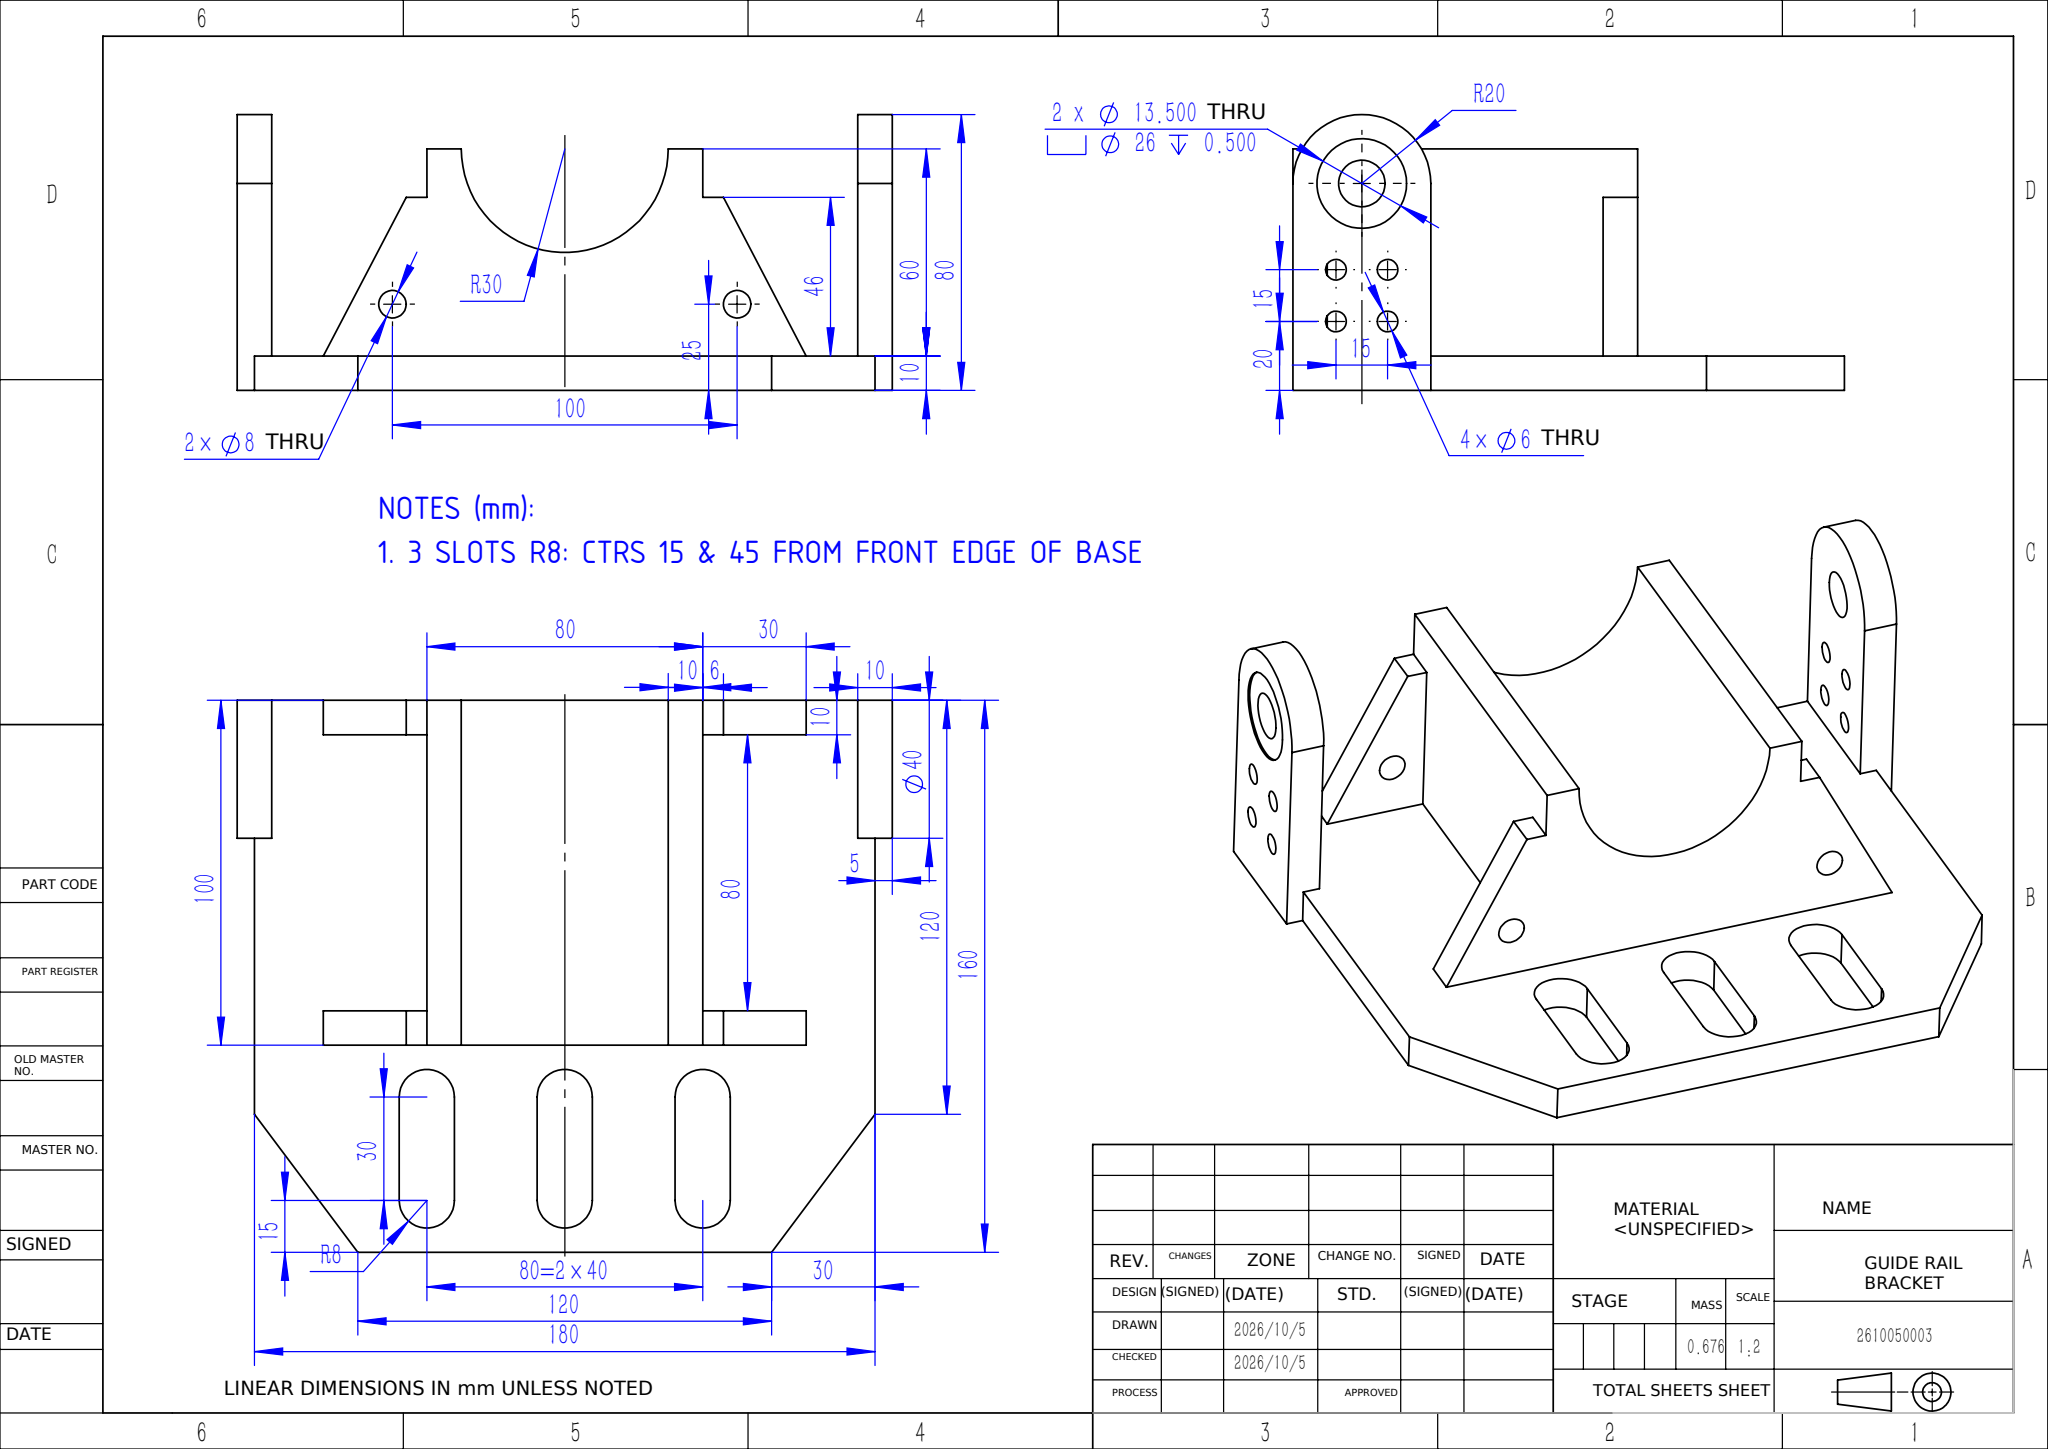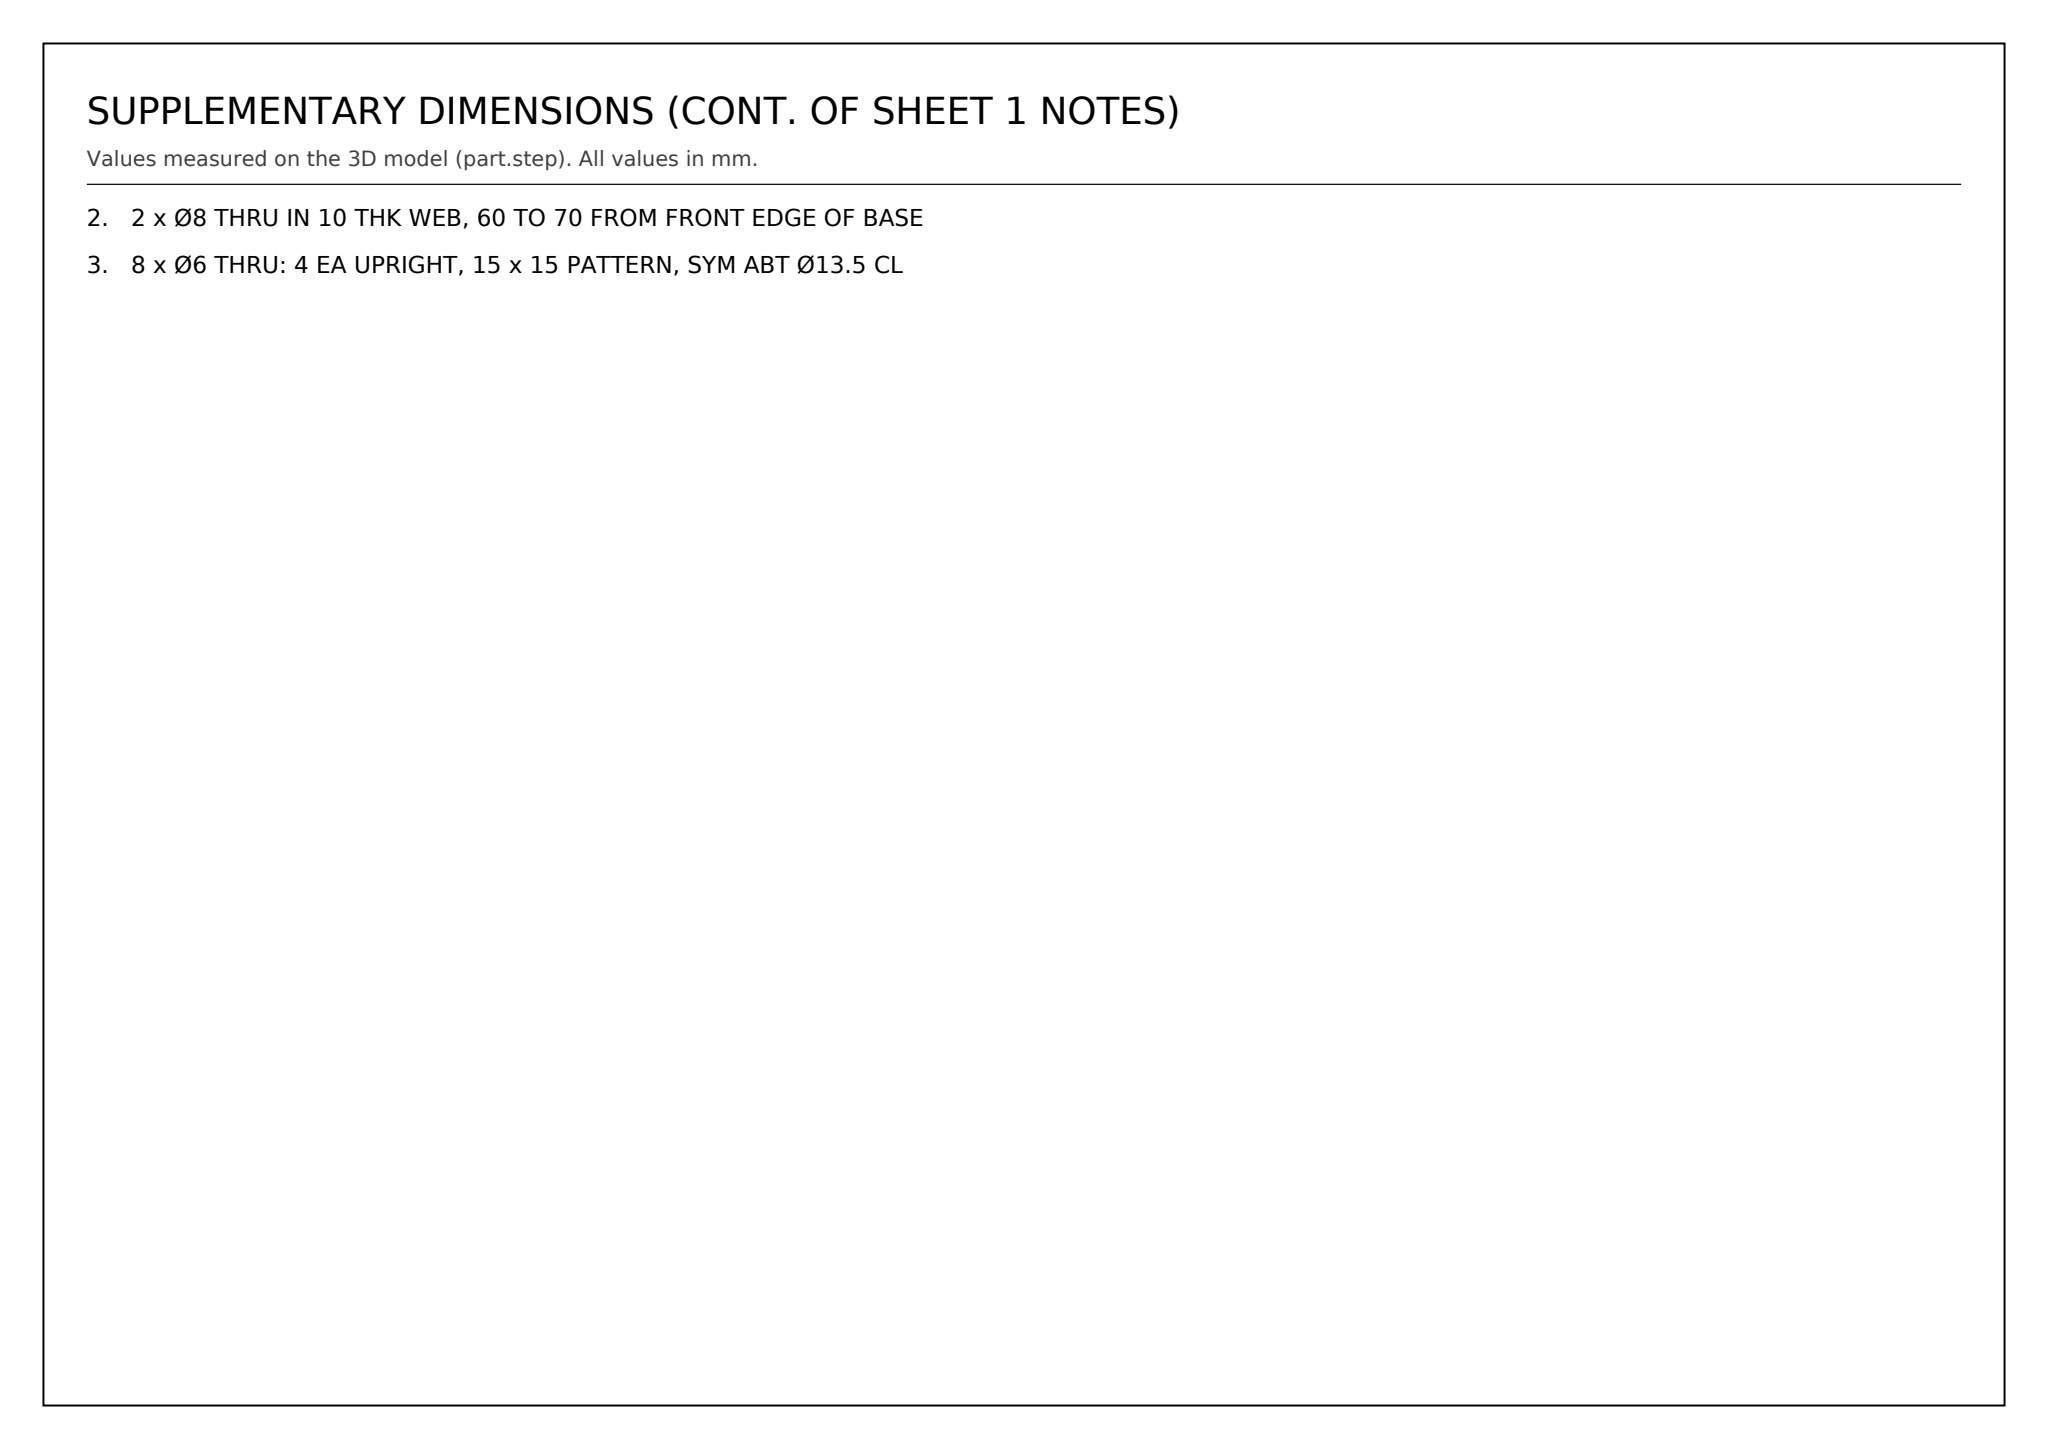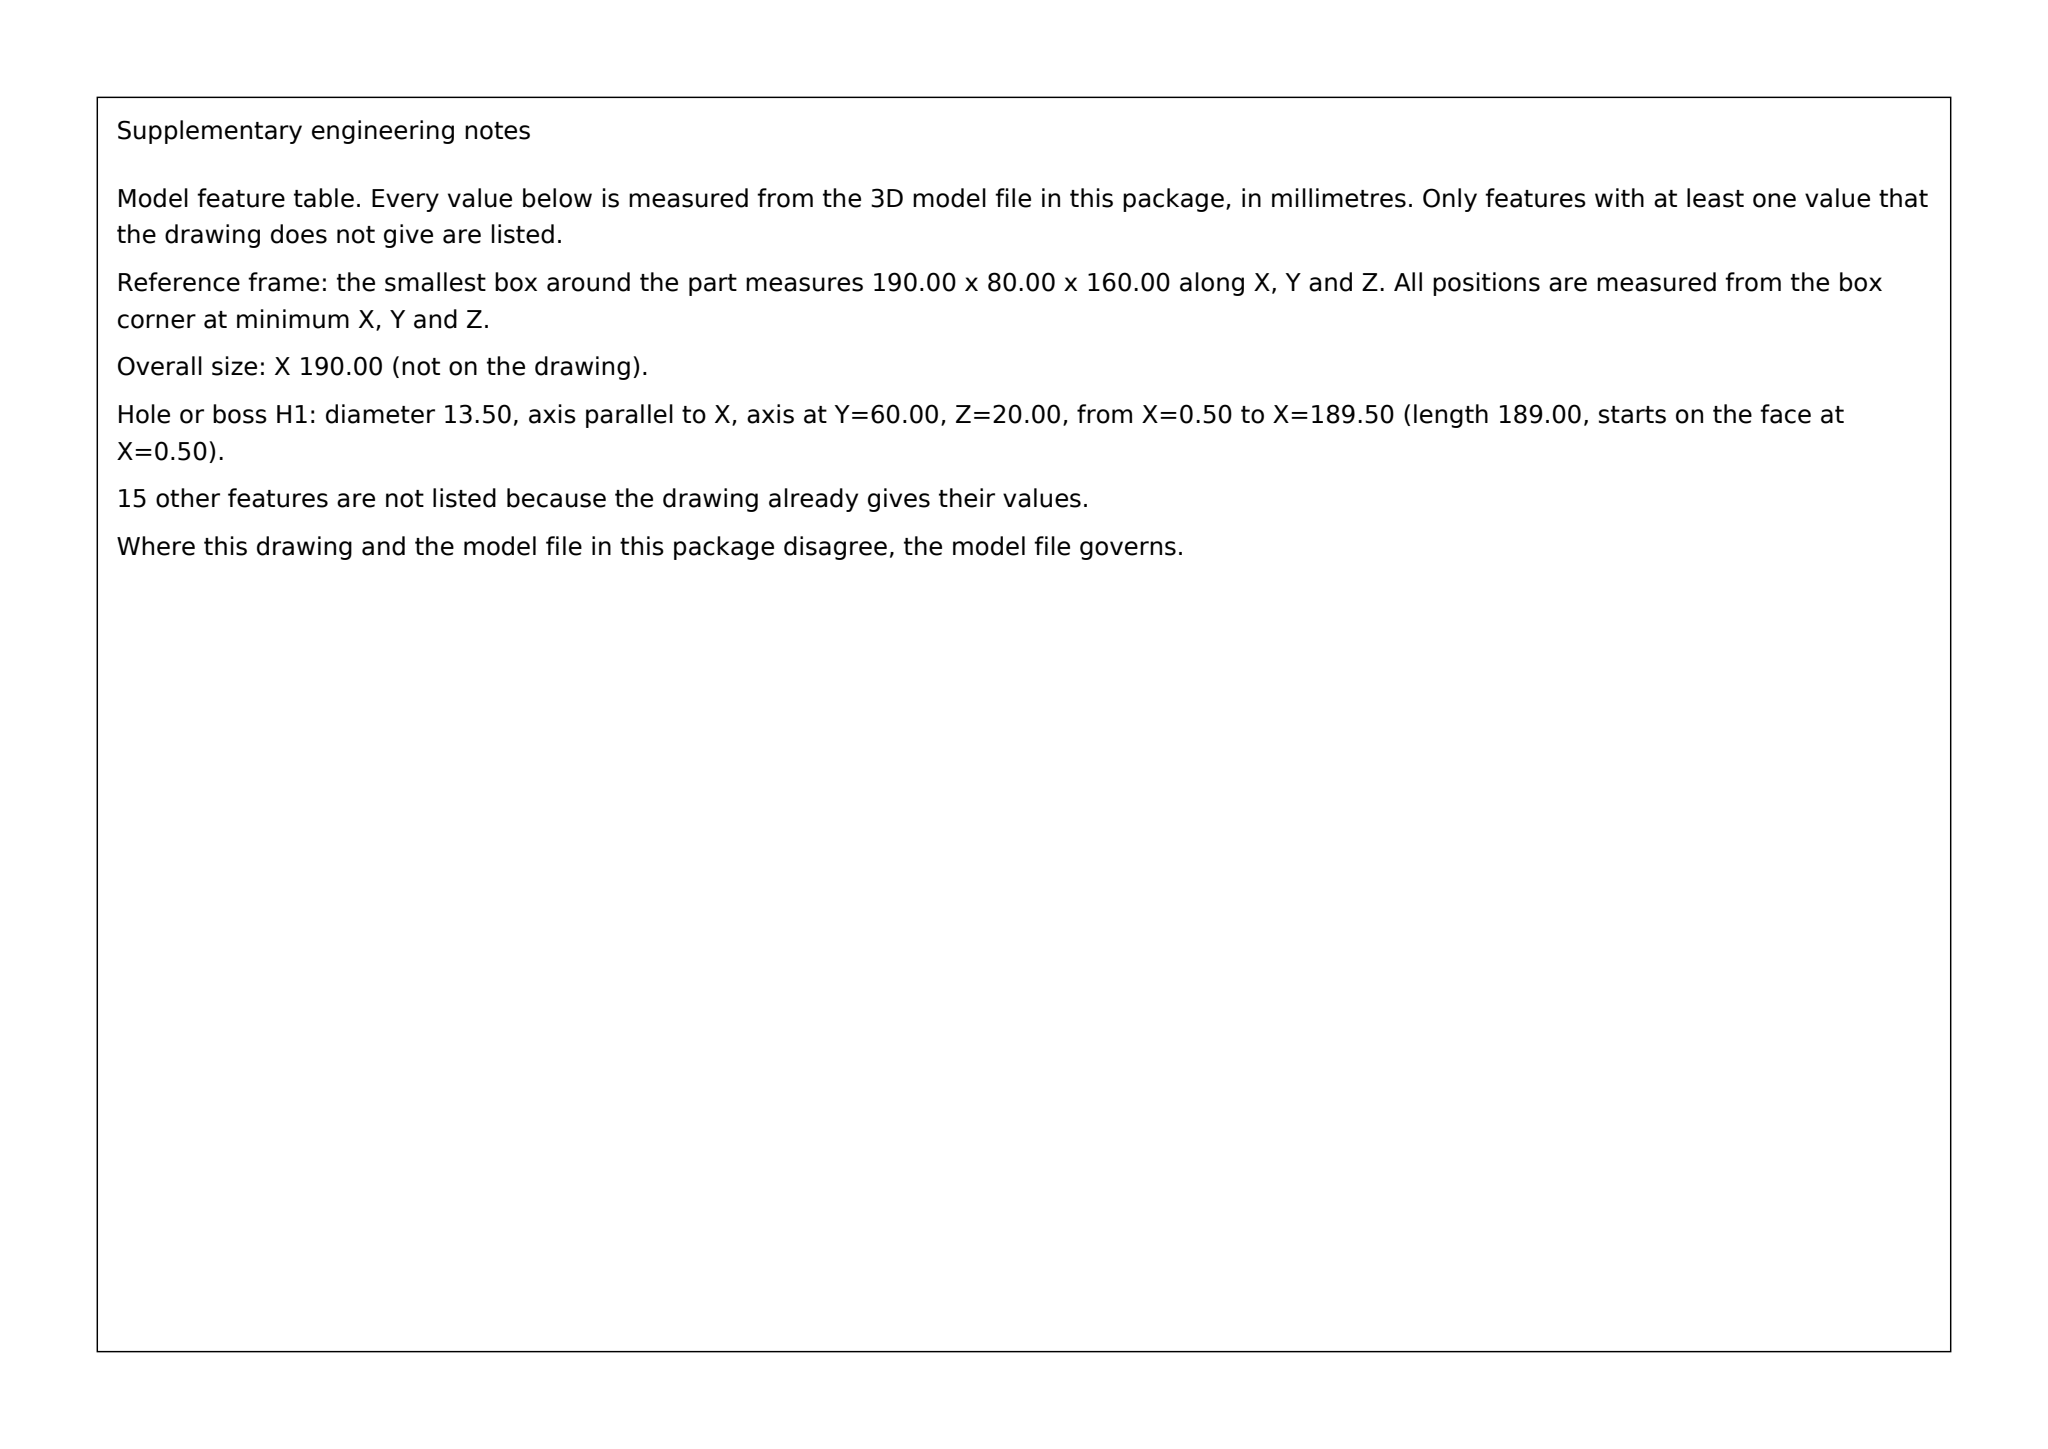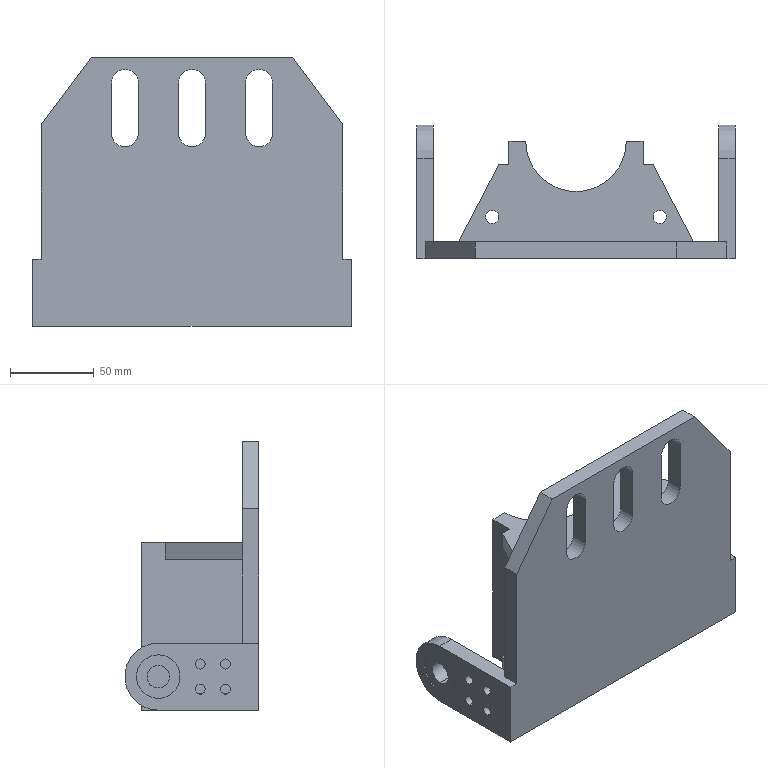Part | SolidWorks | mm | 1 solid | 83 faces | box 190 x 80 x 160 mm | volume 676360 mm3 | cylinder 44 | plane 39 | commonest cylinder face diameters 6 x16 16 x9 8 x8 26 x4 13.5 x4 40 x2 60 x1
Drawing notes:
3 SLOTS R8: CTRS 15 & 45 FROM FRONT EDGE OF BASE | from the solid: Ø16 y-axis cyls at z=115 & 145; base front face z=160 -> 45 & 15
2 x Ø8 THRU IN 10 THK WEB, 60 TO 70 FROM FRONT EDGE OF BASE | from the solid: Ø8 cyls axis z at x=45 & 145, y=25, len 10; web faces z=90 & 100; front edge z=160
8 x Ø6 THRU: 4 EA UPRIGHT, 15 x 15 PATTERN, SYM ABT Ø13.5 CL | from the solid: Ø6 x-axis cyls at y=20/35, z=12.5/27.5, len 10 in plates x=0-10 & 180-190; Ø13.5 axis z=20
build123d program:
from build123d import *

# Parameters (mm, degrees)
BOSS_EXTRUDE1_DEPTH                                  = 10
BOSS_EXTRUDE2_DEPTH                                  = 5
CUT_EXTRUDE1_REACH                                   = 218.852
SKETCH3_R                                            = 3
CYLINDRICAL_COUNTERSUNK_HOLE_FOR_M12_HEX_D           = 13.5
CYLINDRICAL_COUNTERSUNK_HOLE_FOR_M12_HEX_CBORE_D     = 26
CYLINDRICAL_COUNTERSUNK_HOLE_FOR_M12_HEX_CBORE_DEPTH = 0.5
SKETCH7_W                                            = 80
SKETCH7_H                                            = 100
BOSS_EXTRUDE3_DEPTH                                  = 60
CUT_EXTRUDE2_REACH                                   = 161.452
SKETCH8_R                                            = 30
BOSS_EXTRUDE4_DEPTH                                  = 10
SKETCH10_R                                           = 4
CUT_EXTRUDE3_DEPTH                                   = 160.452
CUT_EXTRUDE4_DEPTH                                   = 143.566


with BuildPart() as part:
    # Sketch1 → Boss-Extrude1 (new body)
    with BuildSketch(Plane(origin=(0, 0, 0), x_dir=(1, 0, 0), z_dir=(0, 1, 0))):
        Polygon((-90, -40), (-90, 80), (90, 80), (90, -40), (60, -80), (-60, -80), align=None)
    extrude(amount=BOSS_EXTRUDE1_DEPTH)

    # Sketch2 → Boss-Extrude2 (add, symmetric)
    with BuildSketch(Plane(origin=(90, 0, 0), x_dir=(0, 0, -1), z_dir=(1, 0, 0))):
        with BuildLine():
            Line((80, 0), (40, 0))
            Line((40, 0), (40, 60))
            ThreePointArc((40, 60), (60, 80), (80, 60))
            Line((80, 60), (80, 0))
        make_face()
    boss_extrude2 = extrude(amount=BOSS_EXTRUDE2_DEPTH, both=True)

    # Sketch3 → Cut-Extrude1 (cut, up to next)
    with BuildSketch(Plane(origin=(95, 0, 0), x_dir=(0, 0, -1), z_dir=(1, 0, 0)), mode=Mode.PRIVATE) as cut_extrude1_sk1:
        with Locations((52.5, 35)):
            Circle(SKETCH3_R)
    cut_extrude1_tool1 = extrude(cut_extrude1_sk1.sketch, amount=-CUT_EXTRUDE1_REACH, mode=Mode.PRIVATE) & part.part
    # Sketch3 → Cut-Extrude1 (cut, up to next)
    with BuildSketch(Plane(origin=(95, 0, 0), x_dir=(0, 0, -1), z_dir=(1, 0, 0)), mode=Mode.PRIVATE) as cut_extrude1_sk2:
        with Locations((67.5, 35)):
            Circle(SKETCH3_R)
    cut_extrude1_tool2 = extrude(cut_extrude1_sk2.sketch, amount=-CUT_EXTRUDE1_REACH, mode=Mode.PRIVATE) & part.part
    # Sketch3 → Cut-Extrude1 (cut, up to next)
    with BuildSketch(Plane(origin=(95, 0, 0), x_dir=(0, 0, -1), z_dir=(1, 0, 0)), mode=Mode.PRIVATE) as cut_extrude1_sk3:
        with Locations((52.5, 20)):
            Circle(SKETCH3_R)
    cut_extrude1_tool3 = extrude(cut_extrude1_sk3.sketch, amount=-CUT_EXTRUDE1_REACH, mode=Mode.PRIVATE) & part.part
    # Sketch3 → Cut-Extrude1 (cut, up to next)
    with BuildSketch(Plane(origin=(95, 0, 0), x_dir=(0, 0, -1), z_dir=(1, 0, 0)), mode=Mode.PRIVATE) as cut_extrude1_sk4:
        with Locations((67.5, 20)):
            Circle(SKETCH3_R)
    cut_extrude1_tool4 = extrude(cut_extrude1_sk4.sketch, amount=-CUT_EXTRUDE1_REACH, mode=Mode.PRIVATE) & part.part
    cut_extrude1_1 = cut_extrude1_tool1.solids().sort_by_distance((95, 35, -52.5))[0]
    add(cut_extrude1_1, mode=Mode.SUBTRACT)
    cut_extrude1_2 = cut_extrude1_tool2.solids().sort_by_distance((95, 35, -67.5))[0]
    add(cut_extrude1_2, mode=Mode.SUBTRACT)
    cut_extrude1_3 = cut_extrude1_tool3.solids().sort_by_distance((95, 20, -52.5))[0]
    add(cut_extrude1_3, mode=Mode.SUBTRACT)
    cut_extrude1_4 = cut_extrude1_tool4.solids().sort_by_distance((95, 20, -67.5))[0]
    add(cut_extrude1_4, mode=Mode.SUBTRACT)
    cut_extrude1 = cut_extrude1_1 + cut_extrude1_2 + cut_extrude1_3 + cut_extrude1_4  # Cut-Extrude1 as one shape, for the pattern or mirror that repeats it

    # Cylindrical Countersunk Hole for M12 Hex (through all)
    with Locations(Plane(origin=(95, 0, 0), x_dir=(0, 0, -1), z_dir=(1, 0, 0))):
        with Locations((60, 60)):
            cylindrical_countersunk_hole_for_m12_hex = CounterBoreHole(CYLINDRICAL_COUNTERSUNK_HOLE_FOR_M12_HEX_D / 2, CYLINDRICAL_COUNTERSUNK_HOLE_FOR_M12_HEX_CBORE_D / 2, CYLINDRICAL_COUNTERSUNK_HOLE_FOR_M12_HEX_CBORE_DEPTH)

    # Mirror1: Boss-Extrude2, Cut-Extrude1, Cylindrical Countersunk Hole for M12 Hex across plane
    add(boss_extrude2.mirror(Plane(origin=(0, 0, 0), x_dir=(0, 0, 1), z_dir=(1, 0, 0))))
    add(cut_extrude1.mirror(Plane(origin=(0, 0, 0), x_dir=(0, 0, 1), z_dir=(1, 0, 0))), mode=Mode.SUBTRACT)
    add(cylindrical_countersunk_hole_for_m12_hex.mirror(Plane(origin=(0, 0, 0), x_dir=(0, 0, 1), z_dir=(1, 0, 0))), mode=Mode.SUBTRACT)

    # Sketch7 → Boss-Extrude3 (add)
    with BuildSketch(Plane(origin=(0, 10, 0), x_dir=(1, 0, 0), z_dir=(0, 1, 0))):
        with Locations((0, 30)):
            Rectangle(SKETCH7_W, SKETCH7_H)
    extrude(amount=BOSS_EXTRUDE3_DEPTH)

    # Sketch8 → Cut-Extrude2 (cut, up to next)
    with BuildSketch(Plane.XY.offset(20), mode=Mode.PRIVATE) as cut_extrude2_sk1:
        with Locations((0, 70)):
            Circle(SKETCH8_R)
    cut_extrude2_tool1 = extrude(cut_extrude2_sk1.sketch, amount=-CUT_EXTRUDE2_REACH, mode=Mode.PRIVATE) & part.part
    add(cut_extrude2_tool1.solids().sort_by_distance((0, 70, 20))[0], mode=Mode.SUBTRACT)

    # Sketch9 → Boss-Extrude4 (add)
    with BuildSketch(Plane.XY.offset(20)):
        Polygon((-40, 56), (-46, 56), (-70, 10), (-40, 10), align=None)
        Polygon((40, 56), (46, 56), (70, 10), (40, 10), align=None)
    boss_extrude4 = extrude(amount=-BOSS_EXTRUDE4_DEPTH)

    # Mirror2: Boss-Extrude4 across plane
    add(boss_extrude4.mirror(Plane.XY.offset(-30)))

    # Sketch10 → Cut-Extrude3 (cut, through all)
    with BuildSketch(Plane.XY.offset(20)):
        with Locations((-50, 25)):
            Circle(SKETCH10_R)
        with Locations((50, 25)):
            Circle(SKETCH10_R)
    extrude(amount=-CUT_EXTRUDE3_DEPTH, mode=Mode.SUBTRACT)

    # Sketch11 → Cut-Extrude4 (cut, through all)
    with BuildSketch(Plane(origin=(0, 10, 0), x_dir=(1, 0, 0), z_dir=(0, 1, 0))):
        with BuildLine():
            Line((-32, -35), (-32, -65))
            ThreePointArc((-32, -65), (-40, -73), (-48, -65))
            Line((-48, -65), (-48, -35))
            ThreePointArc((-48, -35), (-40, -27), (-32, -35))
        make_face()
        with BuildLine():
            Line((48, -35), (48, -65))
            ThreePointArc((48, -65), (40, -73), (32, -65))
            Line((32, -65), (32, -35))
            ThreePointArc((32, -35), (40, -27), (48, -35))
        make_face()
        with BuildLine():
            Line((8, -35), (8, -65))
            ThreePointArc((8, -65), (0, -73), (-8, -65))
            Line((-8, -65), (-8, -35))
            ThreePointArc((-8, -35), (0, -27), (8, -35))
        make_face()
    extrude(amount=-CUT_EXTRUDE4_DEPTH, mode=Mode.SUBTRACT)


solid = part.part